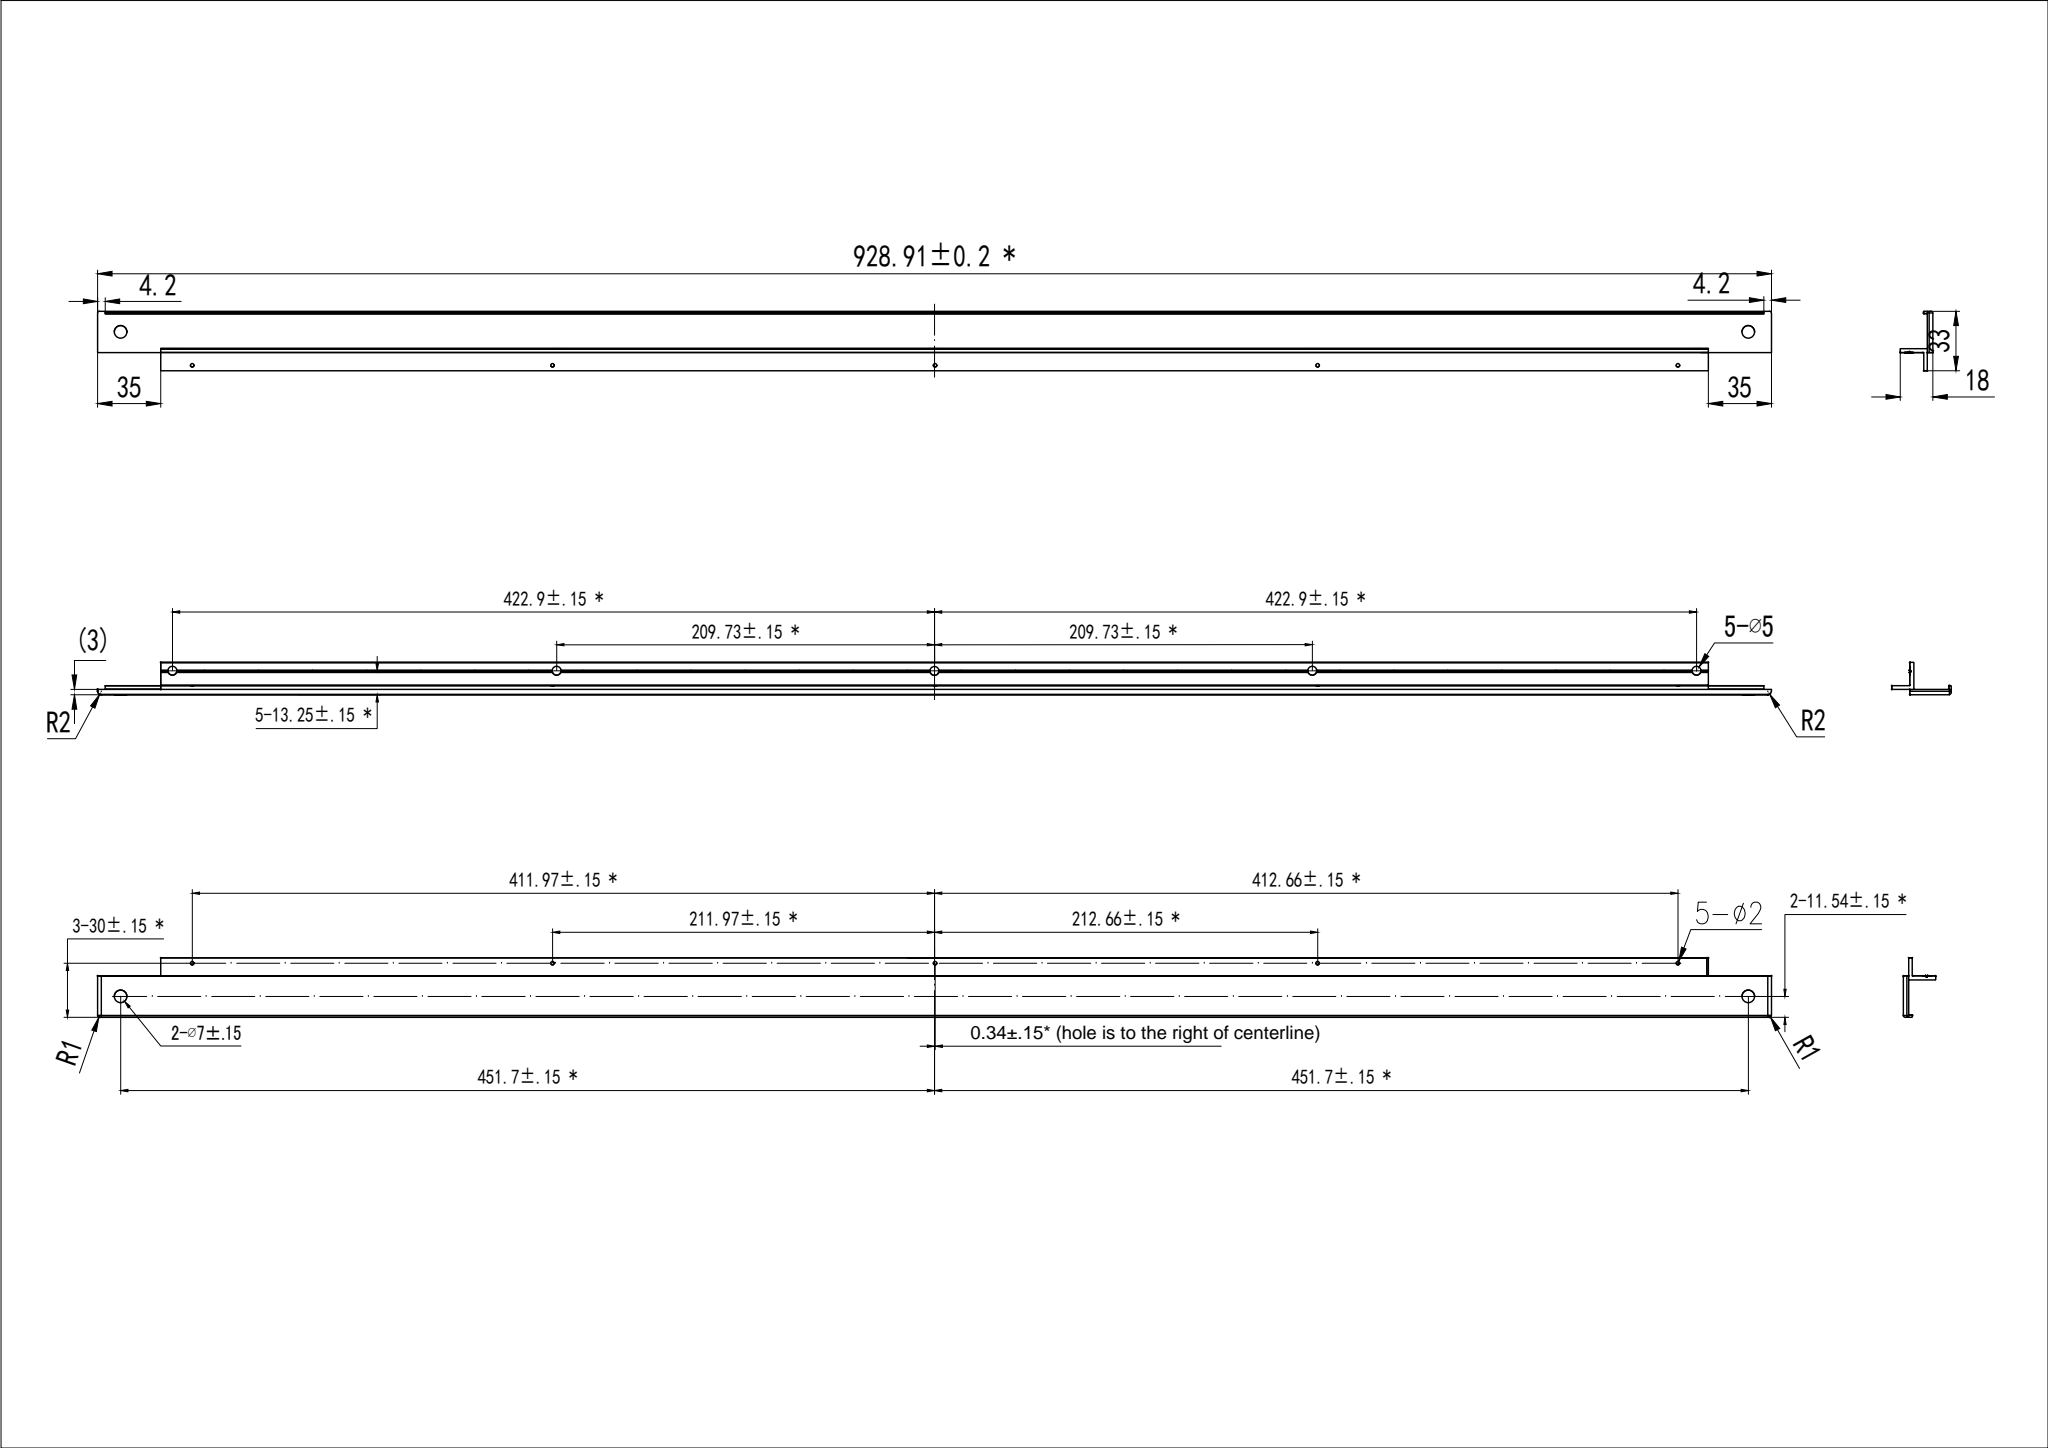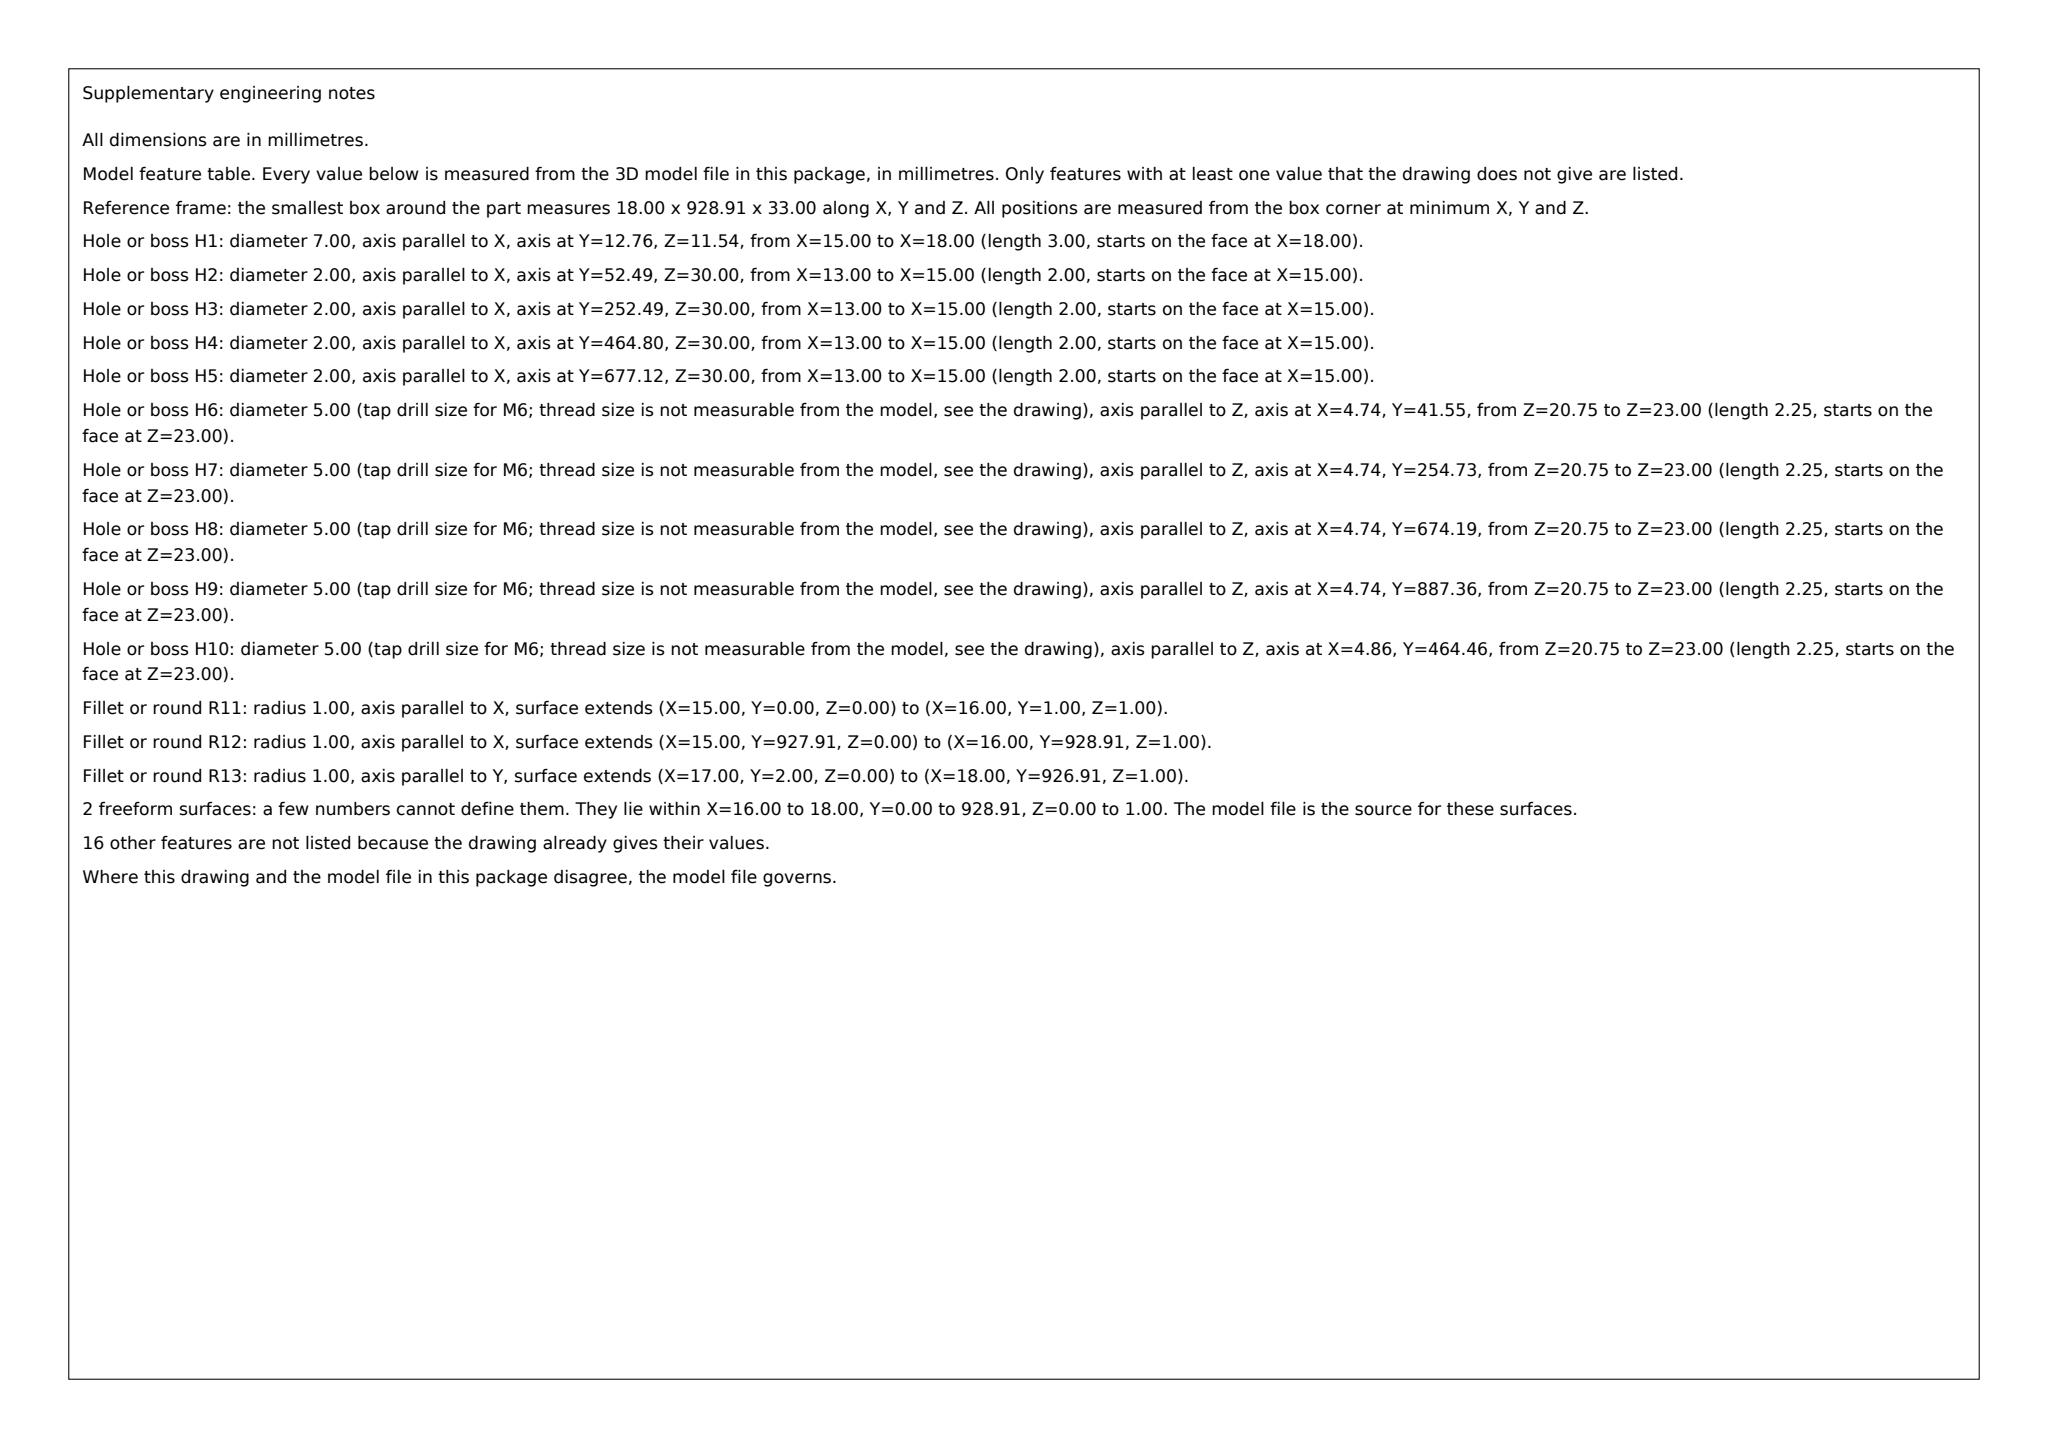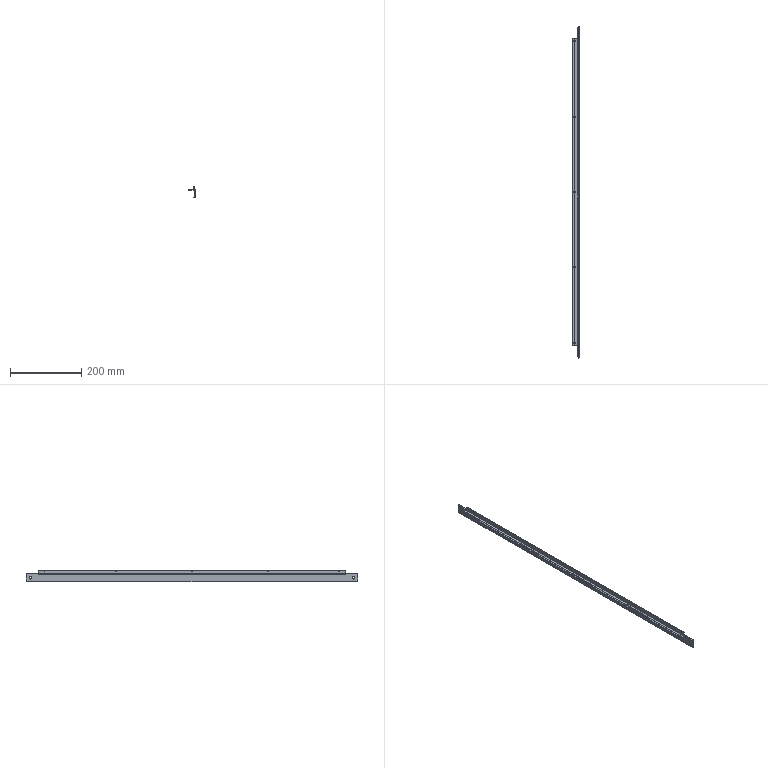Part | SolidWorks | mm | 1 solid | 94 faces | box 18 x 928.91 x 33 mm | volume 111784 mm3 | cylinder 60 | plane 32 | spline 2 | commonest cylinder face diameters 0.4 x30 2 x13 5 x10 7 x4 4 x2 1 x1